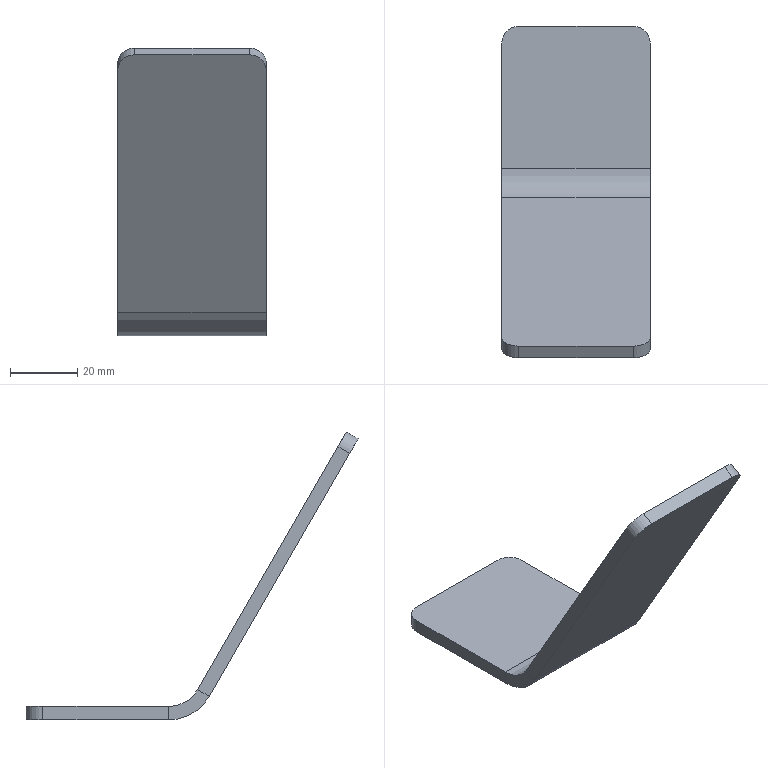Component | SolidWorks | THK-B1015RectangularTubeEndSealingPlate-1 | 1 solid | 18 faces | box 44 x 98.46 x 85.41 mm | volume 25086 mm3 | plane 12 | cylinder 6 | commonest cylinder face diameters 10 x4 28 x1 20 x1 | material Q235A
STEP:
#1=COLOUR_RGB('',0.7922,0.8196,0.9333);
#2=FILL_AREA_STYLE_COLOUR('',#1);
#3=FILL_AREA_STYLE('',(#2));
#4=SURFACE_STYLE_FILL_AREA(#3);
#5=SURFACE_SIDE_STYLE('',(#4));
#6=SURFACE_STYLE_USAGE(.BOTH.,#5);
#7=PRESENTATION_STYLE_ASSIGNMENT((#6));
#8=CARTESIAN_POINT('',(-10.748,-5.678,-35.236));
#9=VERTEX_POINT('',#8);
#10=CARTESIAN_POINT('',(-10.748,-5.678,-35.394));
#11=VERTEX_POINT('',#10);
#12=CARTESIAN_POINT('',(-10.748,-5.678,-35.236));
#13=DIRECTION('',(0.,0.,-1.));
#14=VECTOR('',#13,39.37);
#15=LINE('',#12,#14);
#16=EDGE_CURVE('',#9,#11,#15,.T.);
#17=ORIENTED_EDGE('',*,*,#16,.F.);
#18=CARTESIAN_POINT('',(-10.748,-6.019,-35.039));
#19=VERTEX_POINT('',#18);
#20=CARTESIAN_POINT('',(-10.748,-5.678,-34.843));
#21=DIRECTION('',(-1.,0.,0.));
#22=DIRECTION('',(0.,-1.,0.));
#23=AXIS2_PLACEMENT_3D('',#20,#21,#22);
#24=CIRCLE('',#23,0.3937);
#25=EDGE_CURVE('',#9,#19,#24,.T.);
#26=ORIENTED_EDGE('',*,*,#25,.T.);
#27=CARTESIAN_POINT('',(-10.748,-6.156,-35.118));
#28=VERTEX_POINT('',#27);
#29=CARTESIAN_POINT('',(-10.748,-6.156,-35.118));
#30=DIRECTION('',(0.,0.866,0.5));
#31=VECTOR('',#30,39.37);
#32=LINE('',#29,#31);
#33=EDGE_CURVE('',#28,#19,#32,.T.);
#34=ORIENTED_EDGE('',*,*,#33,.F.);
#35=CARTESIAN_POINT('',(-10.748,-5.678,-34.843));
#36=DIRECTION('',(-1.,0.,0.));
#37=DIRECTION('',(0.,-1.,0.));
#38=AXIS2_PLACEMENT_3D('',#35,#36,#37);
#39=CIRCLE('',#38,0.5512);
#40=EDGE_CURVE('',#11,#28,#39,.T.);
#41=ORIENTED_EDGE('',*,*,#40,.F.);
#42=EDGE_LOOP('',(#17,#26,#34,#41));
#43=FACE_OUTER_BOUND('',#42,.T.);
#44=CARTESIAN_POINT('',(-10.748,-5.678,-35.236));
#45=DIRECTION('',(1.,0.,0.));
#46=DIRECTION('',(0.,-1.,0.));
#47=AXIS2_PLACEMENT_3D('',#44,#45,#46);
#48=PLANE('',#47);
#49=ADVANCED_FACE('',(#43),#48,.T.);
#50=CARTESIAN_POINT('',(-10.748,-4.213,-35.394));
#51=VERTEX_POINT('',#50);
#52=CARTESIAN_POINT('',(-10.748,-4.016,-35.394));
#53=DIRECTION('',(0.,-1.,0.));
#54=VECTOR('',#53,39.37);
#55=LINE('',#52,#54);
#56=EDGE_CURVE('',#51,#11,#55,.T.);
#57=ORIENTED_EDGE('',*,*,#56,.F.);
#58=CARTESIAN_POINT('',(-10.748,-4.213,-35.236));
#59=VERTEX_POINT('',#58);
#60=CARTESIAN_POINT('',(-10.748,-4.213,-35.118));
#61=DIRECTION('',(0.,0.,1.));
#62=VECTOR('',#61,39.37);
#63=LINE('',#60,#62);
#64=EDGE_CURVE('',#51,#59,#63,.T.);
#65=ORIENTED_EDGE('',*,*,#64,.T.);
#66=CARTESIAN_POINT('',(-10.748,-4.016,-35.236));
#67=DIRECTION('',(0.,-1.,0.));
#68=VECTOR('',#67,39.37);
#69=LINE('',#66,#68);
#70=EDGE_CURVE('',#59,#9,#69,.T.);
#71=ORIENTED_EDGE('',*,*,#70,.T.);
#72=ORIENTED_EDGE('',*,*,#16,.T.);
#73=EDGE_LOOP('',(#57,#65,#71,#72));
#74=FACE_OUTER_BOUND('',#73,.T.);
#75=CARTESIAN_POINT('',(-10.748,-6.156,-35.118));
#76=DIRECTION('',(1.,0.,0.));
#77=DIRECTION('',(0.,-1.,0.));
#78=AXIS2_PLACEMENT_3D('',#75,#76,#77);
#79=PLANE('',#78);
#80=ADVANCED_FACE('',(#74),#79,.T.);
#81=CARTESIAN_POINT('',(-12.48,-6.019,-35.039));
#82=VERTEX_POINT('',#81);
#83=CARTESIAN_POINT('',(-12.48,-6.156,-35.118));
#84=VERTEX_POINT('',#83);
#85=CARTESIAN_POINT('',(-12.48,-6.019,-35.039));
#86=DIRECTION('',(0.,-0.866,-0.5));
#87=VECTOR('',#86,39.37);
#88=LINE('',#85,#87);
#89=EDGE_CURVE('',#82,#84,#88,.T.);
#90=ORIENTED_EDGE('',*,*,#89,.F.);
#91=CARTESIAN_POINT('',(-12.48,-5.678,-35.236));
#92=VERTEX_POINT('',#91);
#93=CARTESIAN_POINT('',(-12.48,-5.678,-34.843));
#94=DIRECTION('',(-1.,0.,0.));
#95=DIRECTION('',(0.,-1.,0.));
#96=AXIS2_PLACEMENT_3D('',#93,#94,#95);
#97=CIRCLE('',#96,0.3937);
#98=EDGE_CURVE('',#92,#82,#97,.T.);
#99=ORIENTED_EDGE('',*,*,#98,.F.);
#100=CARTESIAN_POINT('',(-12.48,-5.678,-35.394));
#101=VERTEX_POINT('',#100);
#102=CARTESIAN_POINT('',(-12.48,-5.678,-35.394));
#103=DIRECTION('',(0.,-0.,1.));
#104=VECTOR('',#103,39.37);
#105=LINE('',#102,#104);
#106=EDGE_CURVE('',#101,#92,#105,.T.);
#107=ORIENTED_EDGE('',*,*,#106,.F.);
#108=CARTESIAN_POINT('',(-12.48,-5.678,-34.843));
#109=DIRECTION('',(-1.,0.,0.));
#110=DIRECTION('',(0.,-1.,0.));
#111=AXIS2_PLACEMENT_3D('',#108,#109,#110);
#112=CIRCLE('',#111,0.5512);
#113=EDGE_CURVE('',#101,#84,#112,.T.);
#114=ORIENTED_EDGE('',*,*,#113,.T.);
#115=EDGE_LOOP('',(#90,#99,#107,#114));
#116=FACE_OUTER_BOUND('',#115,.T.);
#117=CARTESIAN_POINT('',(-12.48,-6.019,-35.039));
#118=DIRECTION('',(-1.,0.,0.));
#119=DIRECTION('',(0.,1.,0.));
#120=AXIS2_PLACEMENT_3D('',#117,#118,#119);
#121=PLANE('',#120);
#122=ADVANCED_FACE('',(#116),#121,.T.);
#123=CARTESIAN_POINT('',(-12.48,-7.794,-32.28));
#124=VERTEX_POINT('',#123);
#125=CARTESIAN_POINT('',(-12.48,-6.042,-35.315));
#126=DIRECTION('',(0.,-0.5,0.866));
#127=VECTOR('',#126,39.37);
#128=LINE('',#125,#127);
#129=EDGE_CURVE('',#84,#124,#128,.T.);
#130=ORIENTED_EDGE('',*,*,#129,.T.);
#131=CARTESIAN_POINT('',(-12.48,-7.657,-32.202));
#132=VERTEX_POINT('',#131);
#133=CARTESIAN_POINT('',(-12.48,-7.555,-32.143));
#134=DIRECTION('',(0.,0.866,0.5));
#135=VECTOR('',#134,39.37);
#136=LINE('',#133,#135);
#137=EDGE_CURVE('',#124,#132,#136,.T.);
#138=ORIENTED_EDGE('',*,*,#137,.T.);
#139=CARTESIAN_POINT('',(-12.48,-5.906,-35.236));
#140=DIRECTION('',(0.,-0.5,0.866));
#141=VECTOR('',#140,39.37);
#142=LINE('',#139,#141);
#143=EDGE_CURVE('',#82,#132,#142,.T.);
#144=ORIENTED_EDGE('',*,*,#143,.F.);
#145=ORIENTED_EDGE('',*,*,#89,.T.);
#146=EDGE_LOOP('',(#130,#138,#144,#145));
#147=FACE_OUTER_BOUND('',#146,.T.);
#148=CARTESIAN_POINT('',(-12.48,-5.678,-35.394));
#149=DIRECTION('',(-1.,0.,0.));
#150=DIRECTION('',(0.,1.,0.));
#151=AXIS2_PLACEMENT_3D('',#148,#149,#150);
#152=PLANE('',#151);
#153=ADVANCED_FACE('',(#147),#152,.T.);
#154=ORIENTED_EDGE('',*,*,#143,.T.);
#155=CARTESIAN_POINT('',(-12.283,-7.756,-32.031));
#156=VERTEX_POINT('',#155);
#157=CARTESIAN_POINT('',(-12.283,-7.657,-32.202));
#158=DIRECTION('',(0.,0.866,0.5));
#159=DIRECTION('',(0.,0.5,-0.866));
#160=AXIS2_PLACEMENT_3D('',#157,#158,#159);
#161=CIRCLE('',#160,0.1969);
#162=EDGE_CURVE('',#132,#156,#161,.T.);
#163=ORIENTED_EDGE('',*,*,#162,.T.);
#164=CARTESIAN_POINT('',(-10.945,-7.756,-32.031));
#165=VERTEX_POINT('',#164);
#166=CARTESIAN_POINT('',(-10.748,-7.756,-32.031));
#167=DIRECTION('',(-1.,0.,0.));
#168=VECTOR('',#167,39.37);
#169=LINE('',#166,#168);
#170=EDGE_CURVE('',#165,#156,#169,.T.);
#171=ORIENTED_EDGE('',*,*,#170,.F.);
#172=CARTESIAN_POINT('',(-10.748,-7.657,-32.202));
#173=VERTEX_POINT('',#172);
#174=CARTESIAN_POINT('',(-10.945,-7.657,-32.202));
#175=DIRECTION('',(0.,0.866,0.5));
#176=DIRECTION('',(0.,0.5,-0.866));
#177=AXIS2_PLACEMENT_3D('',#174,#175,#176);
#178=CIRCLE('',#177,0.1969);
#179=EDGE_CURVE('',#165,#173,#178,.T.);
#180=ORIENTED_EDGE('',*,*,#179,.T.);
#181=CARTESIAN_POINT('',(-10.748,-5.906,-35.236));
#182=DIRECTION('',(0.,-0.5,0.866));
#183=VECTOR('',#182,39.37);
#184=LINE('',#181,#183);
#185=EDGE_CURVE('',#19,#173,#184,.T.);
#186=ORIENTED_EDGE('',*,*,#185,.F.);
#187=CARTESIAN_POINT('',(-10.748,-6.019,-35.039));
#188=DIRECTION('',(-1.,0.,0.));
#189=VECTOR('',#188,39.37);
#190=LINE('',#187,#189);
#191=EDGE_CURVE('',#19,#82,#190,.T.);
#192=ORIENTED_EDGE('',*,*,#191,.T.);
#193=EDGE_LOOP('',(#154,#163,#171,#180,#186,#192));
#194=FACE_OUTER_BOUND('',#193,.T.);
#195=CARTESIAN_POINT('',(-10.748,-5.906,-35.236));
#196=DIRECTION('',(0.,-0.866,-0.5));
#197=DIRECTION('',(0.,0.5,-0.866));
#198=AXIS2_PLACEMENT_3D('',#195,#196,#197);
#199=PLANE('',#198);
#200=ADVANCED_FACE('',(#194),#199,.F.);
#201=ORIENTED_EDGE('',*,*,#170,.T.);
#202=CARTESIAN_POINT('',(-12.283,-7.892,-32.11));
#203=VERTEX_POINT('',#202);
#204=CARTESIAN_POINT('',(-12.283,-7.892,-32.11));
#205=DIRECTION('',(0.,-0.866,-0.5));
#206=VECTOR('',#205,39.37);
#207=LINE('',#204,#206);
#208=EDGE_CURVE('',#156,#203,#207,.T.);
#209=ORIENTED_EDGE('',*,*,#208,.T.);
#210=CARTESIAN_POINT('',(-10.945,-7.892,-32.11));
#211=VERTEX_POINT('',#210);
#212=CARTESIAN_POINT('',(-10.748,-7.892,-32.11));
#213=DIRECTION('',(-1.,0.,0.));
#214=VECTOR('',#213,39.37);
#215=LINE('',#212,#214);
#216=EDGE_CURVE('',#211,#203,#215,.T.);
#217=ORIENTED_EDGE('',*,*,#216,.F.);
#218=CARTESIAN_POINT('',(-10.945,-7.892,-32.11));
#219=DIRECTION('',(0.,0.866,0.5));
#220=VECTOR('',#219,39.37);
#221=LINE('',#218,#220);
#222=EDGE_CURVE('',#211,#165,#221,.T.);
#223=ORIENTED_EDGE('',*,*,#222,.T.);
#224=EDGE_LOOP('',(#201,#209,#217,#223));
#225=FACE_OUTER_BOUND('',#224,.T.);
#226=CARTESIAN_POINT('',(-10.748,-7.892,-32.11));
#227=DIRECTION('',(0.,-0.5,0.866));
#228=DIRECTION('',(0.,-0.866,-0.5));
#229=AXIS2_PLACEMENT_3D('',#226,#227,#228);
#230=PLANE('',#229);
#231=ADVANCED_FACE('',(#225),#230,.T.);
#232=ORIENTED_EDGE('',*,*,#216,.T.);
#233=CARTESIAN_POINT('',(-12.283,-7.794,-32.28));
#234=DIRECTION('',(0.,-0.866,-0.5));
#235=DIRECTION('',(0.,0.5,-0.866));
#236=AXIS2_PLACEMENT_3D('',#233,#234,#235);
#237=CIRCLE('',#236,0.1969);
#238=EDGE_CURVE('',#203,#124,#237,.T.);
#239=ORIENTED_EDGE('',*,*,#238,.T.);
#240=ORIENTED_EDGE('',*,*,#129,.F.);
#241=CARTESIAN_POINT('',(-10.748,-6.156,-35.118));
#242=DIRECTION('',(-1.,0.,0.));
#243=VECTOR('',#242,39.37);
#244=LINE('',#241,#243);
#245=EDGE_CURVE('',#28,#84,#244,.T.);
#246=ORIENTED_EDGE('',*,*,#245,.F.);
#247=CARTESIAN_POINT('',(-10.748,-7.794,-32.28));
#248=VERTEX_POINT('',#247);
#249=CARTESIAN_POINT('',(-10.748,-6.042,-35.315));
#250=DIRECTION('',(0.,-0.5,0.866));
#251=VECTOR('',#250,39.37);
#252=LINE('',#249,#251);
#253=EDGE_CURVE('',#28,#248,#252,.T.);
#254=ORIENTED_EDGE('',*,*,#253,.T.);
#255=CARTESIAN_POINT('',(-10.945,-7.794,-32.28));
#256=DIRECTION('',(0.,-0.866,-0.5));
#257=DIRECTION('',(0.,0.5,-0.866));
#258=AXIS2_PLACEMENT_3D('',#255,#256,#257);
#259=CIRCLE('',#258,0.1969);
#260=EDGE_CURVE('',#248,#211,#259,.T.);
#261=ORIENTED_EDGE('',*,*,#260,.T.);
#262=EDGE_LOOP('',(#232,#239,#240,#246,#254,#261));
#263=FACE_OUTER_BOUND('',#262,.T.);
#264=CARTESIAN_POINT('',(-10.748,-6.042,-35.315));
#265=DIRECTION('',(0.,-0.866,-0.5));
#266=DIRECTION('',(0.,0.5,-0.866));
#267=AXIS2_PLACEMENT_3D('',#264,#265,#266);
#268=PLANE('',#267);
#269=ADVANCED_FACE('',(#263),#268,.T.);
#270=ORIENTED_EDGE('',*,*,#113,.F.);
#271=CARTESIAN_POINT('',(-10.748,-5.678,-35.394));
#272=DIRECTION('',(-1.,0.,0.));
#273=VECTOR('',#272,39.37);
#274=LINE('',#271,#273);
#275=EDGE_CURVE('',#11,#101,#274,.T.);
#276=ORIENTED_EDGE('',*,*,#275,.F.);
#277=ORIENTED_EDGE('',*,*,#40,.T.);
#278=ORIENTED_EDGE('',*,*,#245,.T.);
#279=EDGE_LOOP('',(#270,#276,#277,#278));
#280=FACE_OUTER_BOUND('',#279,.T.);
#281=CARTESIAN_POINT('',(-10.748,-5.678,-34.843));
#282=DIRECTION('',(-1.,0.,0.));
#283=DIRECTION('',(0.,1.,0.));
#284=AXIS2_PLACEMENT_3D('',#281,#282,#283);
#285=CYLINDRICAL_SURFACE('',#284,0.5512);
#286=ADVANCED_FACE('',(#280),#285,.T.);
#287=CARTESIAN_POINT('',(-12.48,-4.213,-35.394));
#288=VERTEX_POINT('',#287);
#289=CARTESIAN_POINT('',(-12.48,-4.016,-35.394));
#290=DIRECTION('',(0.,-1.,0.));
#291=VECTOR('',#290,39.37);
#292=LINE('',#289,#291);
#293=EDGE_CURVE('',#288,#101,#292,.T.);
#294=ORIENTED_EDGE('',*,*,#293,.F.);
#295=CARTESIAN_POINT('',(-12.283,-4.016,-35.394));
#296=VERTEX_POINT('',#295);
#297=CARTESIAN_POINT('',(-12.283,-4.213,-35.394));
#298=DIRECTION('',(0.,0.,-1.));
#299=DIRECTION('',(0.,1.,0.));
#300=AXIS2_PLACEMENT_3D('',#297,#298,#299);
#301=CIRCLE('',#300,0.1969);
#302=EDGE_CURVE('',#288,#296,#301,.T.);
#303=ORIENTED_EDGE('',*,*,#302,.T.);
#304=CARTESIAN_POINT('',(-10.945,-4.016,-35.394));
#305=VERTEX_POINT('',#304);
#306=CARTESIAN_POINT('',(-10.748,-4.016,-35.394));
#307=DIRECTION('',(-1.,0.,0.));
#308=VECTOR('',#307,39.37);
#309=LINE('',#306,#308);
#310=EDGE_CURVE('',#305,#296,#309,.T.);
#311=ORIENTED_EDGE('',*,*,#310,.F.);
#312=CARTESIAN_POINT('',(-10.945,-4.213,-35.394));
#313=DIRECTION('',(0.,0.,-1.));
#314=DIRECTION('',(0.,1.,0.));
#315=AXIS2_PLACEMENT_3D('',#312,#313,#314);
#316=CIRCLE('',#315,0.1969);
#317=EDGE_CURVE('',#305,#51,#316,.T.);
#318=ORIENTED_EDGE('',*,*,#317,.T.);
#319=ORIENTED_EDGE('',*,*,#56,.T.);
#320=ORIENTED_EDGE('',*,*,#275,.T.);
#321=EDGE_LOOP('',(#294,#303,#311,#318,#319,#320));
#322=FACE_OUTER_BOUND('',#321,.T.);
#323=CARTESIAN_POINT('',(-10.748,-4.016,-35.394));
#324=DIRECTION('',(0.,0.,-1.));
#325=DIRECTION('',(0.,1.,0.));
#326=AXIS2_PLACEMENT_3D('',#323,#324,#325);
#327=PLANE('',#326);
#328=ADVANCED_FACE('',(#322),#327,.T.);
#329=ORIENTED_EDGE('',*,*,#310,.T.);
#330=CARTESIAN_POINT('',(-12.283,-4.016,-35.236));
#331=VERTEX_POINT('',#330);
#332=CARTESIAN_POINT('',(-12.283,-4.016,-35.236));
#333=DIRECTION('',(0.,0.,1.));
#334=VECTOR('',#333,39.37);
#335=LINE('',#332,#334);
#336=EDGE_CURVE('',#296,#331,#335,.T.);
#337=ORIENTED_EDGE('',*,*,#336,.T.);
#338=CARTESIAN_POINT('',(-10.945,-4.016,-35.236));
#339=VERTEX_POINT('',#338);
#340=CARTESIAN_POINT('',(-10.748,-4.016,-35.236));
#341=DIRECTION('',(-1.,0.,0.));
#342=VECTOR('',#341,39.37);
#343=LINE('',#340,#342);
#344=EDGE_CURVE('',#339,#331,#343,.T.);
#345=ORIENTED_EDGE('',*,*,#344,.F.);
#346=CARTESIAN_POINT('',(-10.945,-4.016,-35.236));
#347=DIRECTION('',(0.,0.,-1.));
#348=VECTOR('',#347,39.37);
#349=LINE('',#346,#348);
#350=EDGE_CURVE('',#339,#305,#349,.T.);
#351=ORIENTED_EDGE('',*,*,#350,.T.);
#352=EDGE_LOOP('',(#329,#337,#345,#351));
#353=FACE_OUTER_BOUND('',#352,.T.);
#354=CARTESIAN_POINT('',(-10.748,-4.016,-35.236));
#355=DIRECTION('',(0.,1.,0.));
#356=DIRECTION('',(1.,0.,0.));
#357=AXIS2_PLACEMENT_3D('',#354,#355,#356);
#358=PLANE('',#357);
#359=ADVANCED_FACE('',(#353),#358,.T.);
#360=ORIENTED_EDGE('',*,*,#344,.T.);
#361=CARTESIAN_POINT('',(-12.48,-4.213,-35.236));
#362=VERTEX_POINT('',#361);
#363=CARTESIAN_POINT('',(-12.283,-4.213,-35.236));
#364=DIRECTION('',(0.,0.,1.));
#365=DIRECTION('',(0.,1.,0.));
#366=AXIS2_PLACEMENT_3D('',#363,#364,#365);
#367=CIRCLE('',#366,0.1969);
#368=EDGE_CURVE('',#331,#362,#367,.T.);
#369=ORIENTED_EDGE('',*,*,#368,.T.);
#370=CARTESIAN_POINT('',(-12.48,-4.016,-35.236));
#371=DIRECTION('',(0.,-1.,0.));
#372=VECTOR('',#371,39.37);
#373=LINE('',#370,#372);
#374=EDGE_CURVE('',#362,#92,#373,.T.);
#375=ORIENTED_EDGE('',*,*,#374,.T.);
#376=CARTESIAN_POINT('',(-10.748,-5.678,-35.236));
#377=DIRECTION('',(-1.,0.,0.));
#378=VECTOR('',#377,39.37);
#379=LINE('',#376,#378);
#380=EDGE_CURVE('',#9,#92,#379,.T.);
#381=ORIENTED_EDGE('',*,*,#380,.F.);
#382=ORIENTED_EDGE('',*,*,#70,.F.);
#383=CARTESIAN_POINT('',(-10.945,-4.213,-35.236));
#384=DIRECTION('',(0.,0.,1.));
#385=DIRECTION('',(0.,1.,0.));
#386=AXIS2_PLACEMENT_3D('',#383,#384,#385);
#387=CIRCLE('',#386,0.1969);
#388=EDGE_CURVE('',#59,#339,#387,.T.);
#389=ORIENTED_EDGE('',*,*,#388,.T.);
#390=EDGE_LOOP('',(#360,#369,#375,#381,#382,#389));
#391=FACE_OUTER_BOUND('',#390,.T.);
#392=CARTESIAN_POINT('',(-10.748,-4.016,-35.236));
#393=DIRECTION('',(0.,0.,-1.));
#394=DIRECTION('',(0.,1.,0.));
#395=AXIS2_PLACEMENT_3D('',#392,#393,#394);
#396=PLANE('',#395);
#397=ADVANCED_FACE('',(#391),#396,.F.);
#398=ORIENTED_EDGE('',*,*,#98,.T.);
#399=ORIENTED_EDGE('',*,*,#191,.F.);
#400=ORIENTED_EDGE('',*,*,#25,.F.);
#401=ORIENTED_EDGE('',*,*,#380,.T.);
#402=EDGE_LOOP('',(#398,#399,#400,#401));
#403=FACE_OUTER_BOUND('',#402,.T.);
#404=CARTESIAN_POINT('',(-10.748,-5.678,-34.843));
#405=DIRECTION('',(-1.,0.,0.));
#406=DIRECTION('',(0.,1.,0.));
#407=AXIS2_PLACEMENT_3D('',#404,#405,#406);
#408=CYLINDRICAL_SURFACE('',#407,0.3937);
#409=ADVANCED_FACE('',(#403),#408,.F.);
#410=ORIENTED_EDGE('',*,*,#185,.T.);
#411=CARTESIAN_POINT('',(-10.748,-7.317,-32.005));
#412=DIRECTION('',(0.,-0.866,-0.5));
#413=VECTOR('',#412,39.37);
#414=LINE('',#411,#413);
#415=EDGE_CURVE('',#173,#248,#414,.T.);
#416=ORIENTED_EDGE('',*,*,#415,.T.);
#417=ORIENTED_EDGE('',*,*,#253,.F.);
#418=ORIENTED_EDGE('',*,*,#33,.T.);
#419=EDGE_LOOP('',(#410,#416,#417,#418));
#420=FACE_OUTER_BOUND('',#419,.T.);
#421=CARTESIAN_POINT('',(-10.748,-5.678,-34.843));
#422=DIRECTION('',(1.,0.,0.));
#423=DIRECTION('',(0.,-1.,0.));
#424=AXIS2_PLACEMENT_3D('',#421,#422,#423);
#425=PLANE('',#424);
#426=ADVANCED_FACE('',(#420),#425,.T.);
#427=ORIENTED_EDGE('',*,*,#374,.F.);
#428=CARTESIAN_POINT('',(-12.48,-4.213,-35.394));
#429=DIRECTION('',(0.,0.,-1.));
#430=VECTOR('',#429,39.37);
#431=LINE('',#428,#430);
#432=EDGE_CURVE('',#362,#288,#431,.T.);
#433=ORIENTED_EDGE('',*,*,#432,.T.);
#434=ORIENTED_EDGE('',*,*,#293,.T.);
#435=ORIENTED_EDGE('',*,*,#106,.T.);
#436=EDGE_LOOP('',(#427,#433,#434,#435));
#437=FACE_OUTER_BOUND('',#436,.T.);
#438=CARTESIAN_POINT('',(-12.48,-5.678,-34.843));
#439=DIRECTION('',(1.,0.,0.));
#440=DIRECTION('',(0.,-1.,0.));
#441=AXIS2_PLACEMENT_3D('',#438,#439,#440);
#442=PLANE('',#441);
#443=ADVANCED_FACE('',(#437),#442,.F.);
#444=ORIENTED_EDGE('',*,*,#238,.F.);
#445=ORIENTED_EDGE('',*,*,#208,.F.);
#446=ORIENTED_EDGE('',*,*,#162,.F.);
#447=ORIENTED_EDGE('',*,*,#137,.F.);
#448=EDGE_LOOP('',(#444,#445,#446,#447));
#449=FACE_OUTER_BOUND('',#448,.T.);
#450=CARTESIAN_POINT('',(-12.283,-7.555,-32.143));
#451=DIRECTION('',(0.,0.866,0.5));
#452=DIRECTION('',(0.,-0.5,0.866));
#453=AXIS2_PLACEMENT_3D('',#450,#451,#452);
#454=CYLINDRICAL_SURFACE('',#453,0.1969);
#455=ADVANCED_FACE('',(#449),#454,.T.);
#456=ORIENTED_EDGE('',*,*,#260,.F.);
#457=ORIENTED_EDGE('',*,*,#415,.F.);
#458=ORIENTED_EDGE('',*,*,#179,.F.);
#459=ORIENTED_EDGE('',*,*,#222,.F.);
#460=EDGE_LOOP('',(#456,#457,#458,#459));
#461=FACE_OUTER_BOUND('',#460,.T.);
#462=CARTESIAN_POINT('',(-10.945,-7.794,-32.28));
#463=DIRECTION('',(0.,0.866,0.5));
#464=DIRECTION('',(0.,-0.5,0.866));
#465=AXIS2_PLACEMENT_3D('',#462,#463,#464);
#466=CYLINDRICAL_SURFACE('',#465,0.1969);
#467=ADVANCED_FACE('',(#461),#466,.T.);
#468=ORIENTED_EDGE('',*,*,#368,.F.);
#469=ORIENTED_EDGE('',*,*,#336,.F.);
#470=ORIENTED_EDGE('',*,*,#302,.F.);
#471=ORIENTED_EDGE('',*,*,#432,.F.);
#472=EDGE_LOOP('',(#468,#469,#470,#471));
#473=FACE_OUTER_BOUND('',#472,.T.);
#474=CARTESIAN_POINT('',(-12.283,-4.213,-34.843));
#475=DIRECTION('',(0.,0.,1.));
#476=DIRECTION('',(0.,-1.,0.));
#477=AXIS2_PLACEMENT_3D('',#474,#475,#476);
#478=CYLINDRICAL_SURFACE('',#477,0.1969);
#479=ADVANCED_FACE('',(#473),#478,.T.);
#480=ORIENTED_EDGE('',*,*,#388,.F.);
#481=ORIENTED_EDGE('',*,*,#64,.F.);
#482=ORIENTED_EDGE('',*,*,#317,.F.);
#483=ORIENTED_EDGE('',*,*,#350,.F.);
#484=EDGE_LOOP('',(#480,#481,#482,#483));
#485=FACE_OUTER_BOUND('',#484,.T.);
#486=CARTESIAN_POINT('',(-10.945,-4.213,-35.236));
#487=DIRECTION('',(0.,0.,-1.));
#488=DIRECTION('',(0.,1.,0.));
#489=AXIS2_PLACEMENT_3D('',#486,#487,#488);
#490=CYLINDRICAL_SURFACE('',#489,0.1969);
#491=ADVANCED_FACE('',(#485),#490,.T.);
#492=CLOSED_SHELL('',(#49,#80,#122,#153,#200,#231,#269,#286,#328,#359,#397,#409,#426,#443,#455,#467,#479,#491));
#493=MANIFOLD_SOLID_BREP('',#492);
#494=STYLED_ITEM('',(#7),#493);
#495=PRESENTATION_LAYER_ASSIGNMENT('','',(#494));
#496=(LENGTH_UNIT()NAMED_UNIT(*)SI_UNIT($,.METRE.));
#497=LENGTH_MEASURE_WITH_UNIT(LENGTH_MEASURE(0.0254),#496);
#498=DIMENSIONAL_EXPONENTS(1.,0.,0.,0.,0.,0.,0.);
#499=(CONVERSION_BASED_UNIT('',#497)LENGTH_UNIT()NAMED_UNIT(#498));
#500=UNCERTAINTY_MEASURE_WITH_UNIT(LENGTH_MEASURE(0.00001),#499,'','');
#501=(NAMED_UNIT(*)PLANE_ANGLE_UNIT()SI_UNIT($,.RADIAN.));
#502=(NAMED_UNIT(*)SI_UNIT($,.STERADIAN.)SOLID_ANGLE_UNIT());
#503=(GEOMETRIC_REPRESENTATION_CONTEXT(3)GLOBAL_UNCERTAINTY_ASSIGNED_CONTEXT((#500))GLOBAL_UNIT_ASSIGNED_CONTEXT((#499,#501,#502))REPRESENTATION_CONTEXT('',''));
#504=MECHANICAL_DESIGN_GEOMETRIC_PRESENTATION_REPRESENTATION('',(#494),#503);
#505=CARTESIAN_POINT('',(0.,0.,0.));
#506=DIRECTION('',(0.,0.,1.));
#507=DIRECTION('',(1.,0.,0.));
#508=AXIS2_PLACEMENT_3D('',#505,#506,#507);
#509=(LENGTH_UNIT()NAMED_UNIT(*)SI_UNIT($,.METRE.));
#510=LENGTH_MEASURE_WITH_UNIT(LENGTH_MEASURE(0.0254),#509);
#511=DIMENSIONAL_EXPONENTS(1.,0.,0.,0.,0.,0.,0.);
#512=(CONVERSION_BASED_UNIT('',#510)LENGTH_UNIT()NAMED_UNIT(#511));
#513=UNCERTAINTY_MEASURE_WITH_UNIT(LENGTH_MEASURE(0.00001),#512,'','');
#514=(NAMED_UNIT(*)PLANE_ANGLE_UNIT()SI_UNIT($,.RADIAN.));
#515=(NAMED_UNIT(*)SI_UNIT($,.STERADIAN.)SOLID_ANGLE_UNIT());
#516=(GEOMETRIC_REPRESENTATION_CONTEXT(3)GLOBAL_UNCERTAINTY_ASSIGNED_CONTEXT((#513))GLOBAL_UNIT_ASSIGNED_CONTEXT((#512,#514,#515))REPRESENTATION_CONTEXT('',''));
#517=ADVANCED_BREP_SHAPE_REPRESENTATION('',(#493,#508),#516);